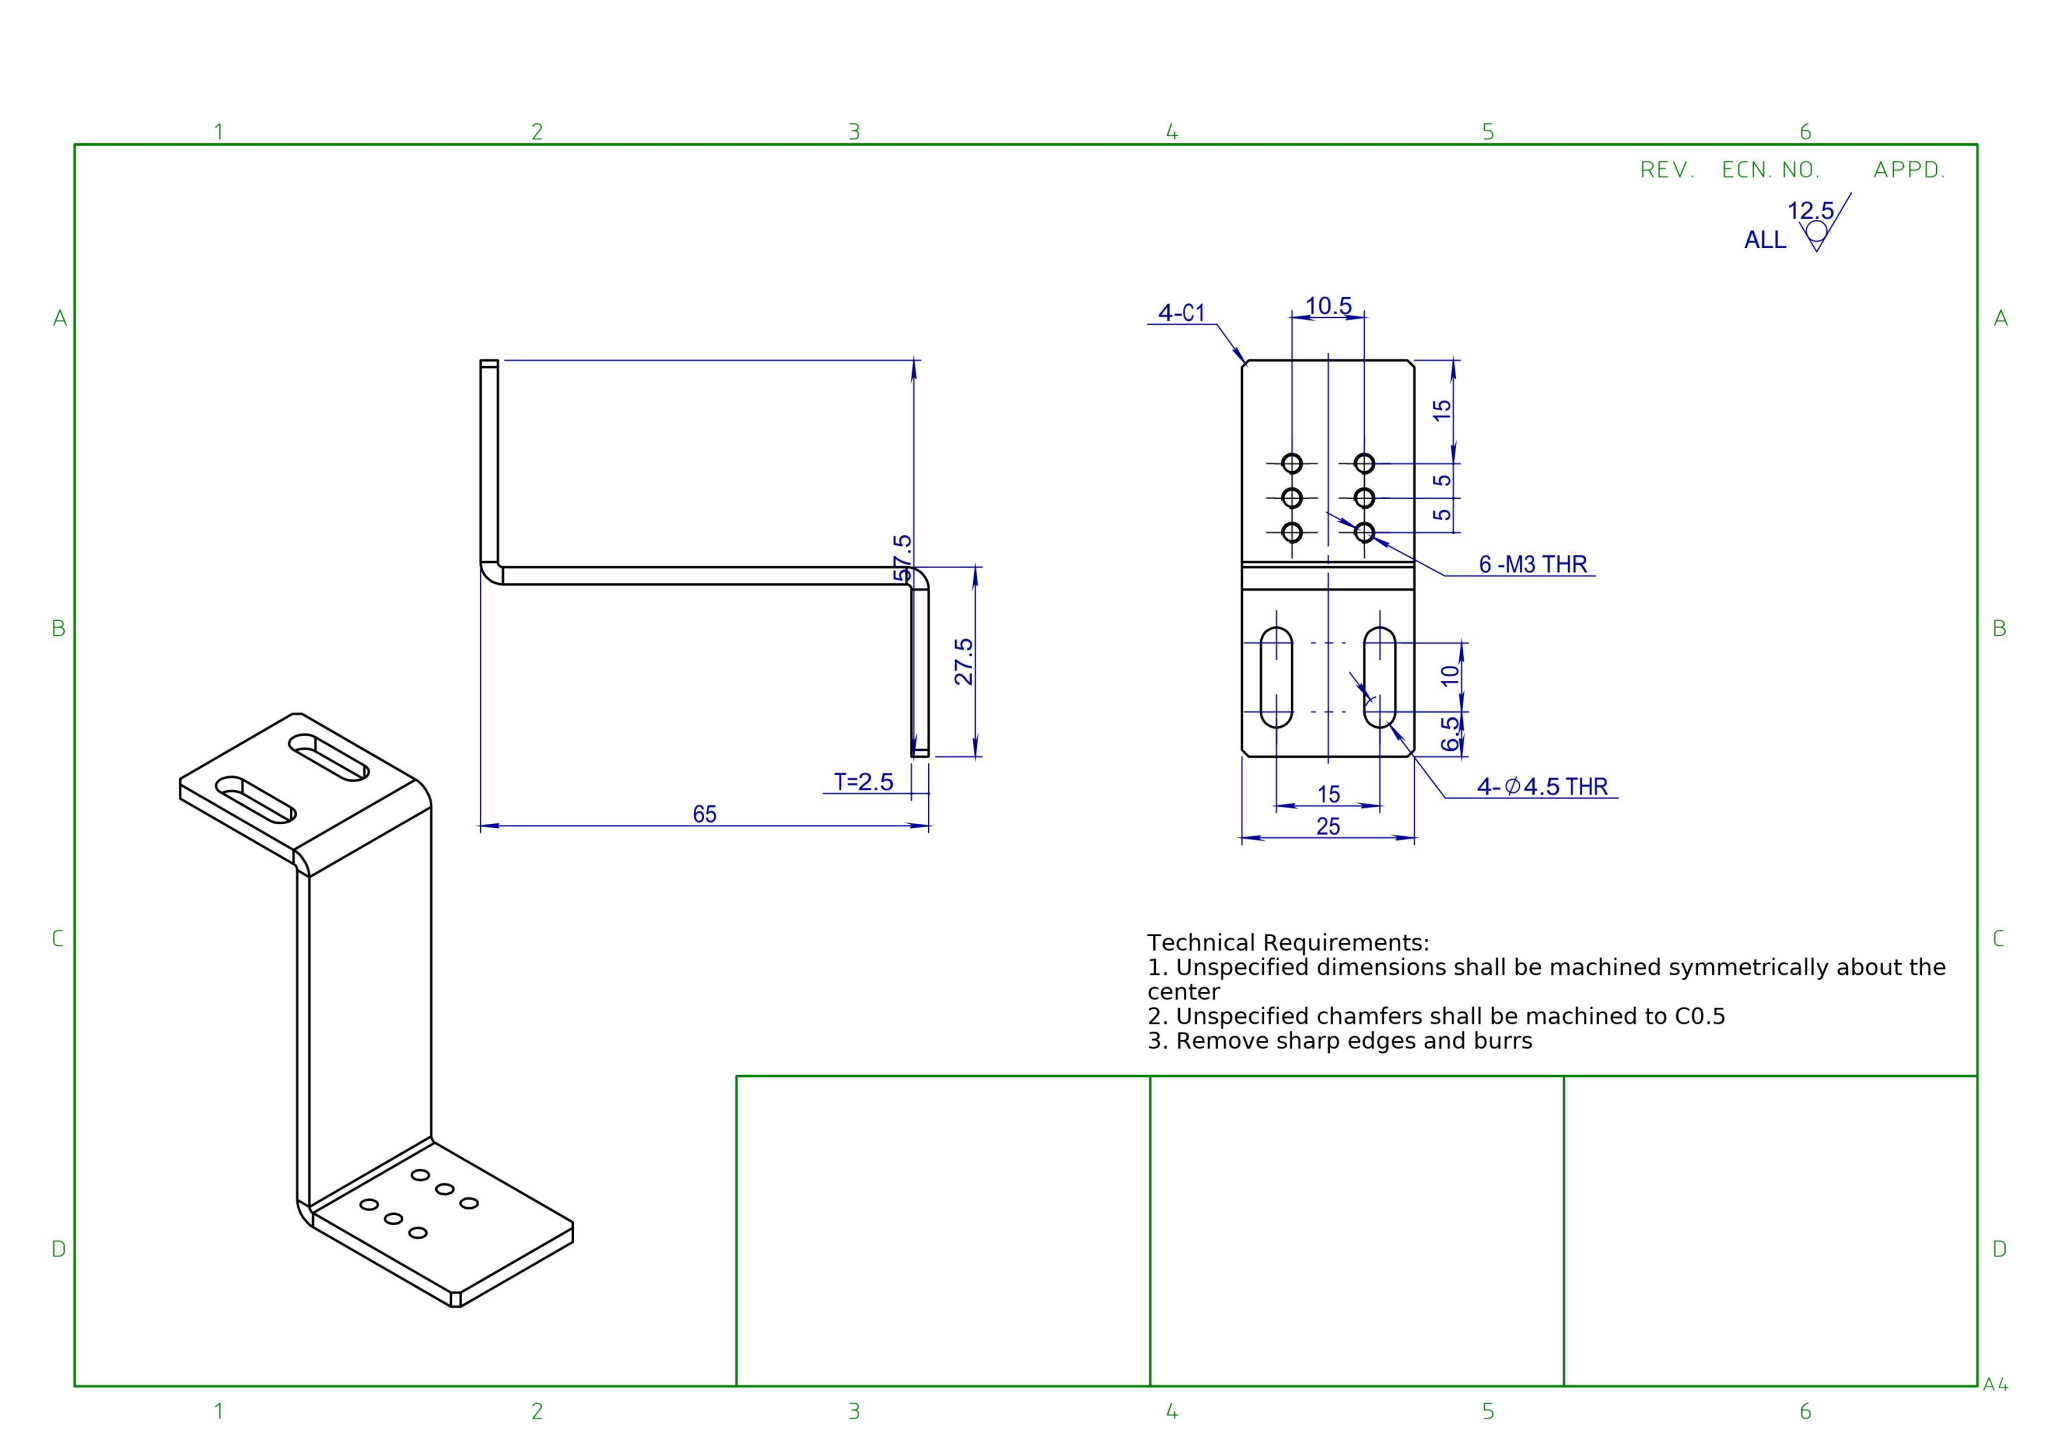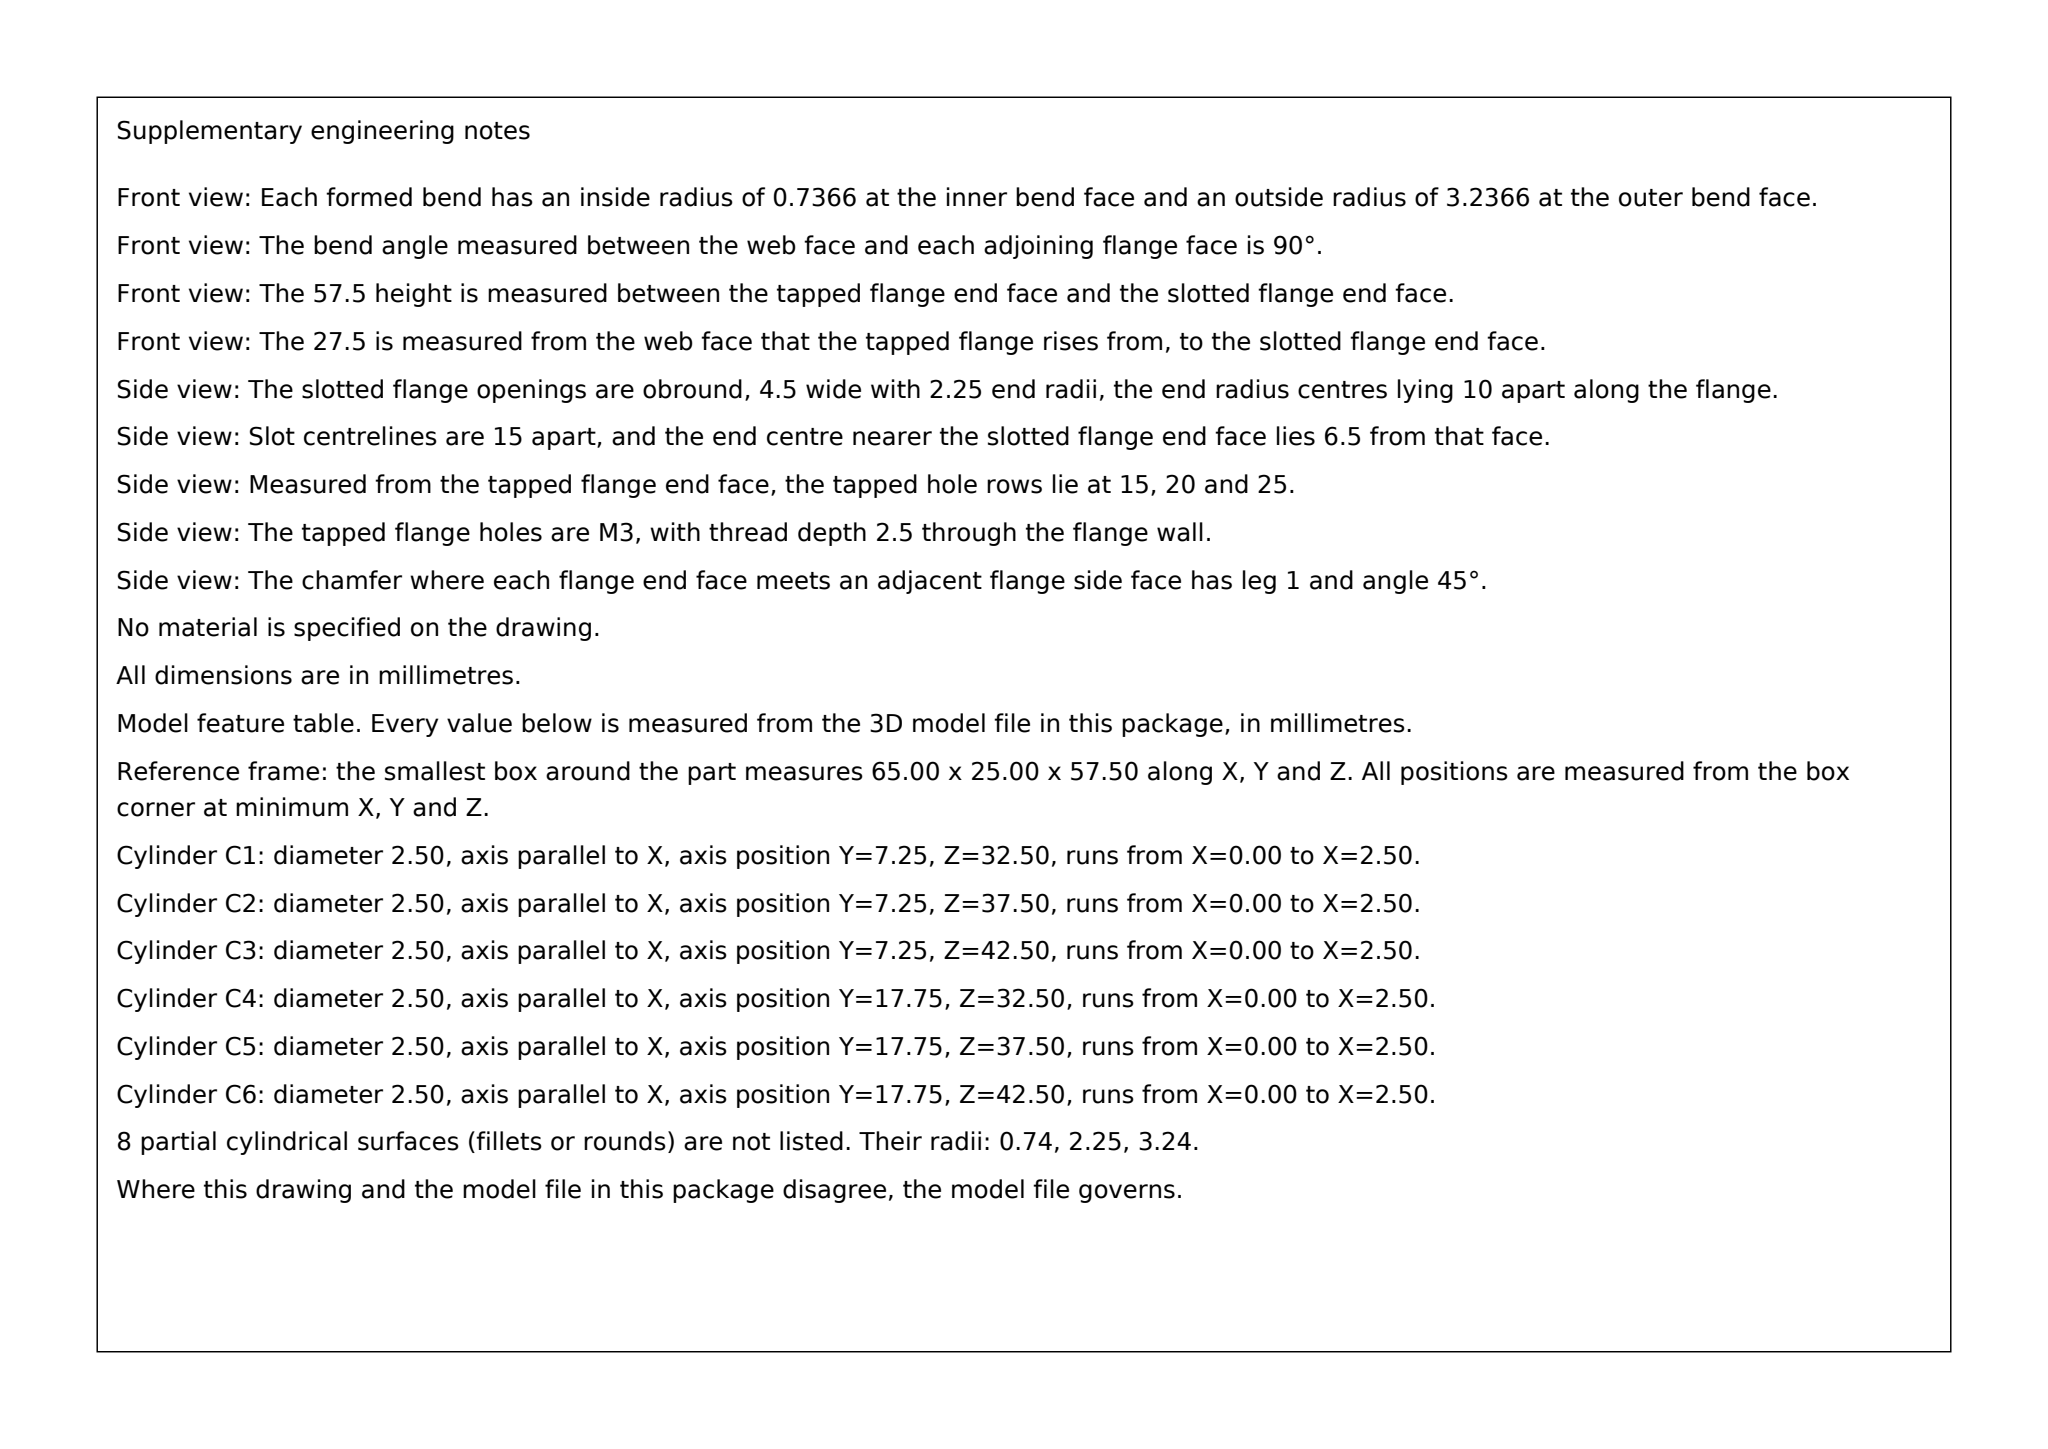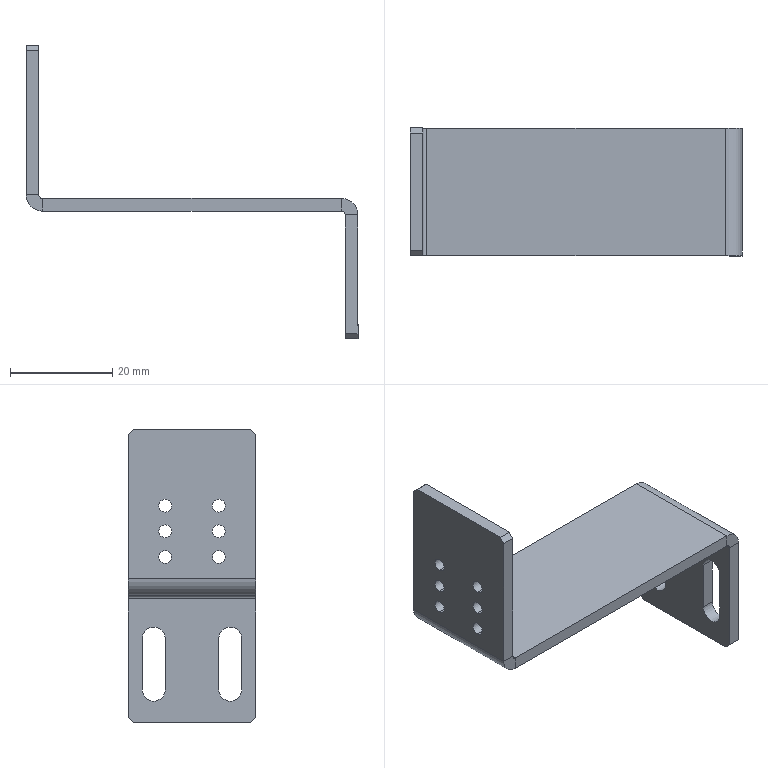Part | SolidWorks | mm | 1 solid | 48 faces | box 65 x 25 x 57.5 mm | volume 7010 mm3 | plane 26 | cylinder 22 | commonest cylinder face diameters 2.5 x12 4.5 x6 6.473 x2 1.473 x2